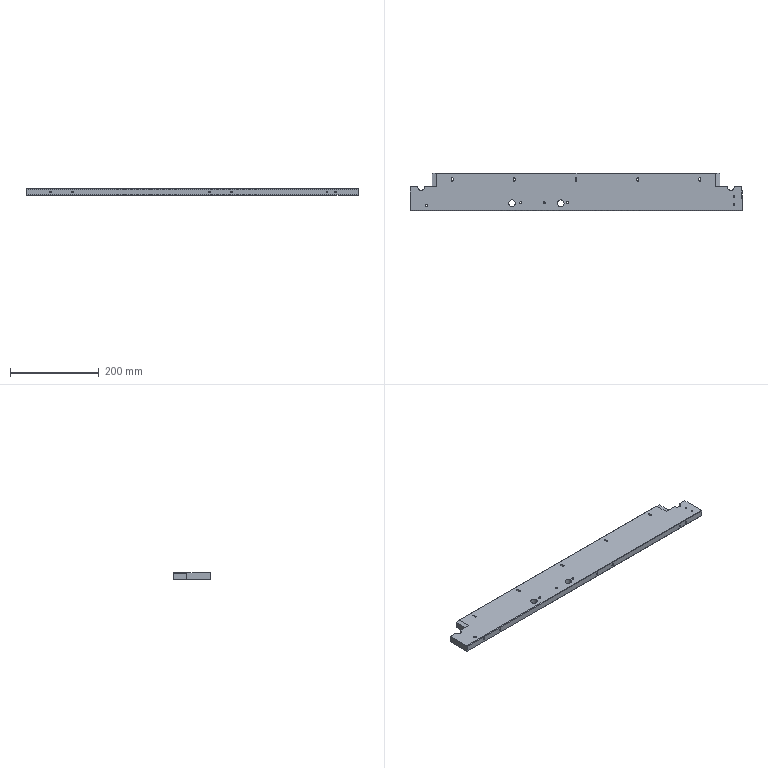Component | SolidWorks | XT-1-02-2-1 | 1 solid | 131 faces | box 750 x 85 x 15 mm | volume 884214 mm3 | cylinder 62 | plane 49 | cone 20 | commonest cylinder face diameters 4.2 x20 4.5 x10 8 x10 5 x6 15 x6 3.3 x4 4 x4 6 x2
build123d program:
from build123d import *

# Parameters (mm, degrees)
SKETCH1_W                                       = 750
SKETCH1_H                                       = 85
BOSS_EXTRUDE1_DEPTH                             = 15
SKETCH2_R                                       = 7.5
SKETCH2_W                                       = 50
SKETCH2_H                                       = 31
CUT_EXTRUDE1_DEPTH                              = 755.95
SKETCH3_R                                       = 7.5
CUT_EXTRUDE2_DEPTH                              = 755.95
M5_TAPPED_HOLE1_D                               = 4.2
M5_TAPPED_HOLE1_DEPTH                           = 15
M5_TAPPED_HOLE1_TIP                             = 1.262
SKETCH6_W                                       = 30
SKETCH6_H                                       = 30
CUT_EXTRUDE3_DEPTH                              = 8
M6_TAPPED_HOLE1_D                               = 5
M4_HEX_SOCKET_HEAD_CAP_SCREW_CBORE1_D           = 4.5
M4_HEX_SOCKET_HEAD_CAP_SCREW_CBORE1_CBORE_D     = 8
M4_HEX_SOCKET_HEAD_CAP_SCREW_CBORE1_CBORE_DEPTH = 4.4
CUT_EXTRUDE4_DEPTH                              = 755.95
CUT_EXTRUDE5_DEPTH                              = 7
M5_TAPPED_HOLE2_D                               = 4.2
M5_TAPPED_HOLE2_DEPTH                           = 15
M5_TAPPED_HOLE2_TIP                             = 1.262
F_6_0_6_DIAMETER_HOLE1_D                        = 6
SKETCH21_R                                      = 2
CUT_EXTRUDE6_DEPTH                              = 8
CHAMFER1_SIZE                                   = 1
CHAMFER2_SIZE                                   = 10
CHAMFER2_SIZE2                                  = 2
CHAMFER3_SIZE                                   = 1
M4_TAPPED_HOLE1_D                               = 3.3
M4_TAPPED_HOLE1_DEPTH                           = 10.1
M4_TAPPED_HOLE1_TIP                             = 0.9914


with BuildPart() as part:
    # Sketch1 → Boss-Extrude1 (new body)
    with BuildSketch(Plane.XY):
        with Locations((375, -42.5)):
            Rectangle(SKETCH1_W, SKETCH1_H)
    extrude(amount=BOSS_EXTRUDE1_DEPTH)

    # Sketch2 → Cut-Extrude1 (cut, through all)
    with BuildSketch(Plane.XY.offset(15)):
        with Locations((230.5, -68)):
            Circle(SKETCH2_R)
        with Locations((340.5, -68)):
            Circle(SKETCH2_R)
        with Locations((25, -15.5)):
            Rectangle(SKETCH2_W, SKETCH2_H)
        with Locations((725, -15.5)):
            Rectangle(SKETCH2_W, SKETCH2_H)
    extrude(amount=-CUT_EXTRUDE1_DEPTH, mode=Mode.SUBTRACT)

    # Sketch3 → Cut-Extrude2 (cut, through all)
    with BuildSketch(Plane.XY.offset(15)):
        with Locations((25, -31)):
            Circle(SKETCH3_R)
        with Locations((725, -31)):
            Circle(SKETCH3_R)
    extrude(amount=-CUT_EXTRUDE2_DEPTH, mode=Mode.SUBTRACT)

    # M5 Tapped Hole1
    with Locations(Plane(origin=(0, -31, 0), x_dir=(1, 0, 0), z_dir=(0, 1, 0))):
        with Locations((9.5, -7.5), (40.5, -7.5), (709.5, -7.5), (740.5, -7.5)):
            Hole(M5_TAPPED_HOLE1_D / 2, depth=M5_TAPPED_HOLE1_DEPTH)
            with Locations((0, 0, -(M5_TAPPED_HOLE1_DEPTH + M5_TAPPED_HOLE1_TIP / 2))):  # 118° drill point
                Cone(0, M5_TAPPED_HOLE1_D / 2, M5_TAPPED_HOLE1_TIP, mode=Mode.SUBTRACT)

    # Sketch6 → Cut-Extrude3 (cut)
    with BuildSketch(Plane(origin=(0, 0, 0), x_dir=(-1, 0, 0), z_dir=(0, 0, -1))):
        with Locations((-735, -62)):
            Rectangle(SKETCH6_W, SKETCH6_H)
    extrude(amount=-CUT_EXTRUDE3_DEPTH, mode=Mode.SUBTRACT)

    # M6 Tapped Hole1 (through all)
    with Locations(Plane(origin=(0, 0, 0), x_dir=(-1, 0, 0), z_dir=(0, 0, -1))):
        with Locations((-250, -67), (-303, -67), (-356, -67)):
            Hole(M6_TAPPED_HOLE1_D / 2)

    # M4 Hex Socket Head Cap Screw CBORE1 (through all)
    with Locations(Plane(origin=(0, 0, 0), x_dir=(-1, 0, 0), z_dir=(0, 0, -1))):
        with Locations((-95, -14), (-235, -14), (-375, -14), (-515, -14), (-655, -14)):
            CounterBoreHole(M4_HEX_SOCKET_HEAD_CAP_SCREW_CBORE1_D / 2, M4_HEX_SOCKET_HEAD_CAP_SCREW_CBORE1_CBORE_D / 2, M4_HEX_SOCKET_HEAD_CAP_SCREW_CBORE1_CBORE_DEPTH)

    # Sketch11 → Cut-Extrude4 (cut, through all)
    with BuildSketch(Plane(origin=(0, 0, 0), x_dir=(-1, 0, 0), z_dir=(0, 0, -1))):
        with BuildLine():
            Line((-652.75, -11.5), (-652.75, -16.5))
            ThreePointArc((-652.75, -16.5), (-655, -18.75), (-657.25, -16.5))
            Line((-657.25, -16.5), (-657.25, -11.5))
            ThreePointArc((-657.25, -11.5), (-655, -9.25), (-652.75, -11.5))
        make_face()
        with BuildLine():
            Line((-512.75, -11.5), (-512.75, -16.5))
            ThreePointArc((-512.75, -16.5), (-515, -18.75), (-517.25, -16.5))
            Line((-517.25, -16.5), (-517.25, -11.5))
            ThreePointArc((-517.25, -11.5), (-515, -9.25), (-512.75, -11.5))
        make_face()
        with BuildLine():
            Line((-372.75, -11.5), (-372.75, -16.5))
            ThreePointArc((-372.75, -16.5), (-375, -18.75), (-377.25, -16.5))
            Line((-377.25, -16.5), (-377.25, -11.5))
            ThreePointArc((-377.25, -11.5), (-375, -9.25), (-372.75, -11.5))
        make_face()
        with BuildLine():
            Line((-232.75, -11.5), (-232.75, -16.5))
            ThreePointArc((-232.75, -16.5), (-235, -18.75), (-237.25, -16.5))
            Line((-237.25, -16.5), (-237.25, -11.5))
            ThreePointArc((-237.25, -11.5), (-235, -9.25), (-232.75, -11.5))
        make_face()
        with BuildLine():
            Line((-92.75, -11.5), (-92.75, -16.5))
            ThreePointArc((-92.75, -16.5), (-95, -18.75), (-97.25, -16.5))
            Line((-97.25, -16.5), (-97.25, -11.5))
            ThreePointArc((-97.25, -11.5), (-95, -9.25), (-92.75, -11.5))
        make_face()
    extrude(amount=-CUT_EXTRUDE4_DEPTH, mode=Mode.SUBTRACT)

    # Sketch12 → Cut-Extrude5 (cut)
    with BuildSketch(Plane(origin=(0, 0, 0), x_dir=(-1, 0, 0), z_dir=(0, 0, -1))):
        with BuildLine():
            Line((-651, -11.5), (-651, -16.5))
            ThreePointArc((-651, -16.5), (-655, -20.5), (-659, -16.5))
            Line((-659, -16.5), (-659, -11.5))
            ThreePointArc((-659, -11.5), (-655, -7.5), (-651, -11.5))
        make_face()
        with BuildLine():
            Line((-511, -11.5), (-511, -16.5))
            ThreePointArc((-511, -16.5), (-515, -20.5), (-519, -16.5))
            Line((-519, -16.5), (-519, -11.5))
            ThreePointArc((-519, -11.5), (-515, -7.5), (-511, -11.5))
        make_face()
        with BuildLine():
            Line((-379, -16.5), (-379, -11.5))
            ThreePointArc((-379, -11.5), (-375, -7.5), (-371, -11.5))
            Line((-371, -11.5), (-371, -16.5))
            ThreePointArc((-371, -16.5), (-375, -20.5), (-379, -16.5))
        make_face()
        with BuildLine():
            Line((-239, -16.5), (-239, -11.5))
            ThreePointArc((-239, -11.5), (-235, -7.5), (-231, -11.5))
            Line((-231, -11.5), (-231, -16.5))
            ThreePointArc((-231, -16.5), (-235, -20.5), (-239, -16.5))
        make_face()
        with BuildLine():
            Line((-99, -16.5), (-99, -11.5))
            ThreePointArc((-99, -11.5), (-95, -7.5), (-91, -11.5))
            Line((-91, -11.5), (-91, -16.5))
            ThreePointArc((-91, -16.5), (-95, -20.5), (-99, -16.5))
        make_face()
    extrude(amount=-CUT_EXTRUDE5_DEPTH, mode=Mode.SUBTRACT)

    # M5 Tapped Hole2
    with Locations(Plane(origin=(0, -85, 0), x_dir=(-1, 0, 0), z_dir=(0, -1, 0))):
        with Locations((-680, -7.5), (-700, -7.5), (-465, -7.5), (-415, -7.5), (-105, -7.5), (-55, -7.5)):
            Hole(M5_TAPPED_HOLE2_D / 2, depth=M5_TAPPED_HOLE2_DEPTH)
            with Locations((0, 0, -(M5_TAPPED_HOLE2_DEPTH + M5_TAPPED_HOLE2_TIP / 2))):  # 118° drill point
                Cone(0, M5_TAPPED_HOLE2_D / 2, M5_TAPPED_HOLE2_TIP, mode=Mode.SUBTRACT)

    # 6.0 _6_ Diameter Hole1 (through all)
    with Locations(Plane(origin=(0, 0, 0), x_dir=(-1, 0, 0), z_dir=(0, 0, -1))):
        with Locations((-37, -73)):
            Hole(F_6_0_6_DIAMETER_HOLE1_D / 2)

    # Sketch21 → Cut-Extrude6 (cut)
    with BuildSketch(Plane(origin=(0, 0, 0), x_dir=(-1, 0, 0), z_dir=(0, 0, -1))):
        with Locations((-720, -49)):
            Circle(SKETCH21_R)
        with Locations((-720, -75)):
            Circle(SKETCH21_R)
    extrude(amount=-CUT_EXTRUDE6_DEPTH, mode=Mode.SUBTRACT)

    # Chamfer1
    chamfer1_edges = [part.edges().sort_by_distance(p)[0] for p in [
        (375, 0, 0),
        (375, 0, 15),
        (375, -85, 0),
        (375, -85, 15),
    ]]
    chamfer(chamfer1_edges, length=CHAMFER1_SIZE)

    # Chamfer2
    chamfer2_edges = [part.edges().sort_by_distance(p)[0] for p in [
        (50, -16, 15),
        (700, -16, 15),
    ]]
    chamfer2_side = [part.faces().sort_by_distance(p)[0] for p in [
        (375.777, -43.785, 15),
    ]]
    chamfer(chamfer2_edges, length=CHAMFER2_SIZE, length2=CHAMFER2_SIZE2, reference=chamfer2_side[0])

    # Chamfer3
    chamfer3_edges = [part.edges().sort_by_distance(p)[0] for p in [
        (700, 0, 7),
        (50, 0, 7),
    ]]
    chamfer(chamfer3_edges, length=CHAMFER3_SIZE)

    # M4 Tapped Hole1
    with Locations(Plane(origin=(0, 0, 8), x_dir=(-1, 0, 0), z_dir=(0, 0, -1))):
        with Locations((-732, -53), (-732, -71)):
            Hole(M4_TAPPED_HOLE1_D / 2, depth=M4_TAPPED_HOLE1_DEPTH)
            with Locations((0, 0, -(M4_TAPPED_HOLE1_DEPTH + M4_TAPPED_HOLE1_TIP / 2))):  # 118° drill point
                Cone(0, M4_TAPPED_HOLE1_D / 2, M4_TAPPED_HOLE1_TIP, mode=Mode.SUBTRACT)


solid = part.part

# Placed as in the assembly
solid = solid.moved(Location((214.283, 139.385, -153), (0, 0, 0)))